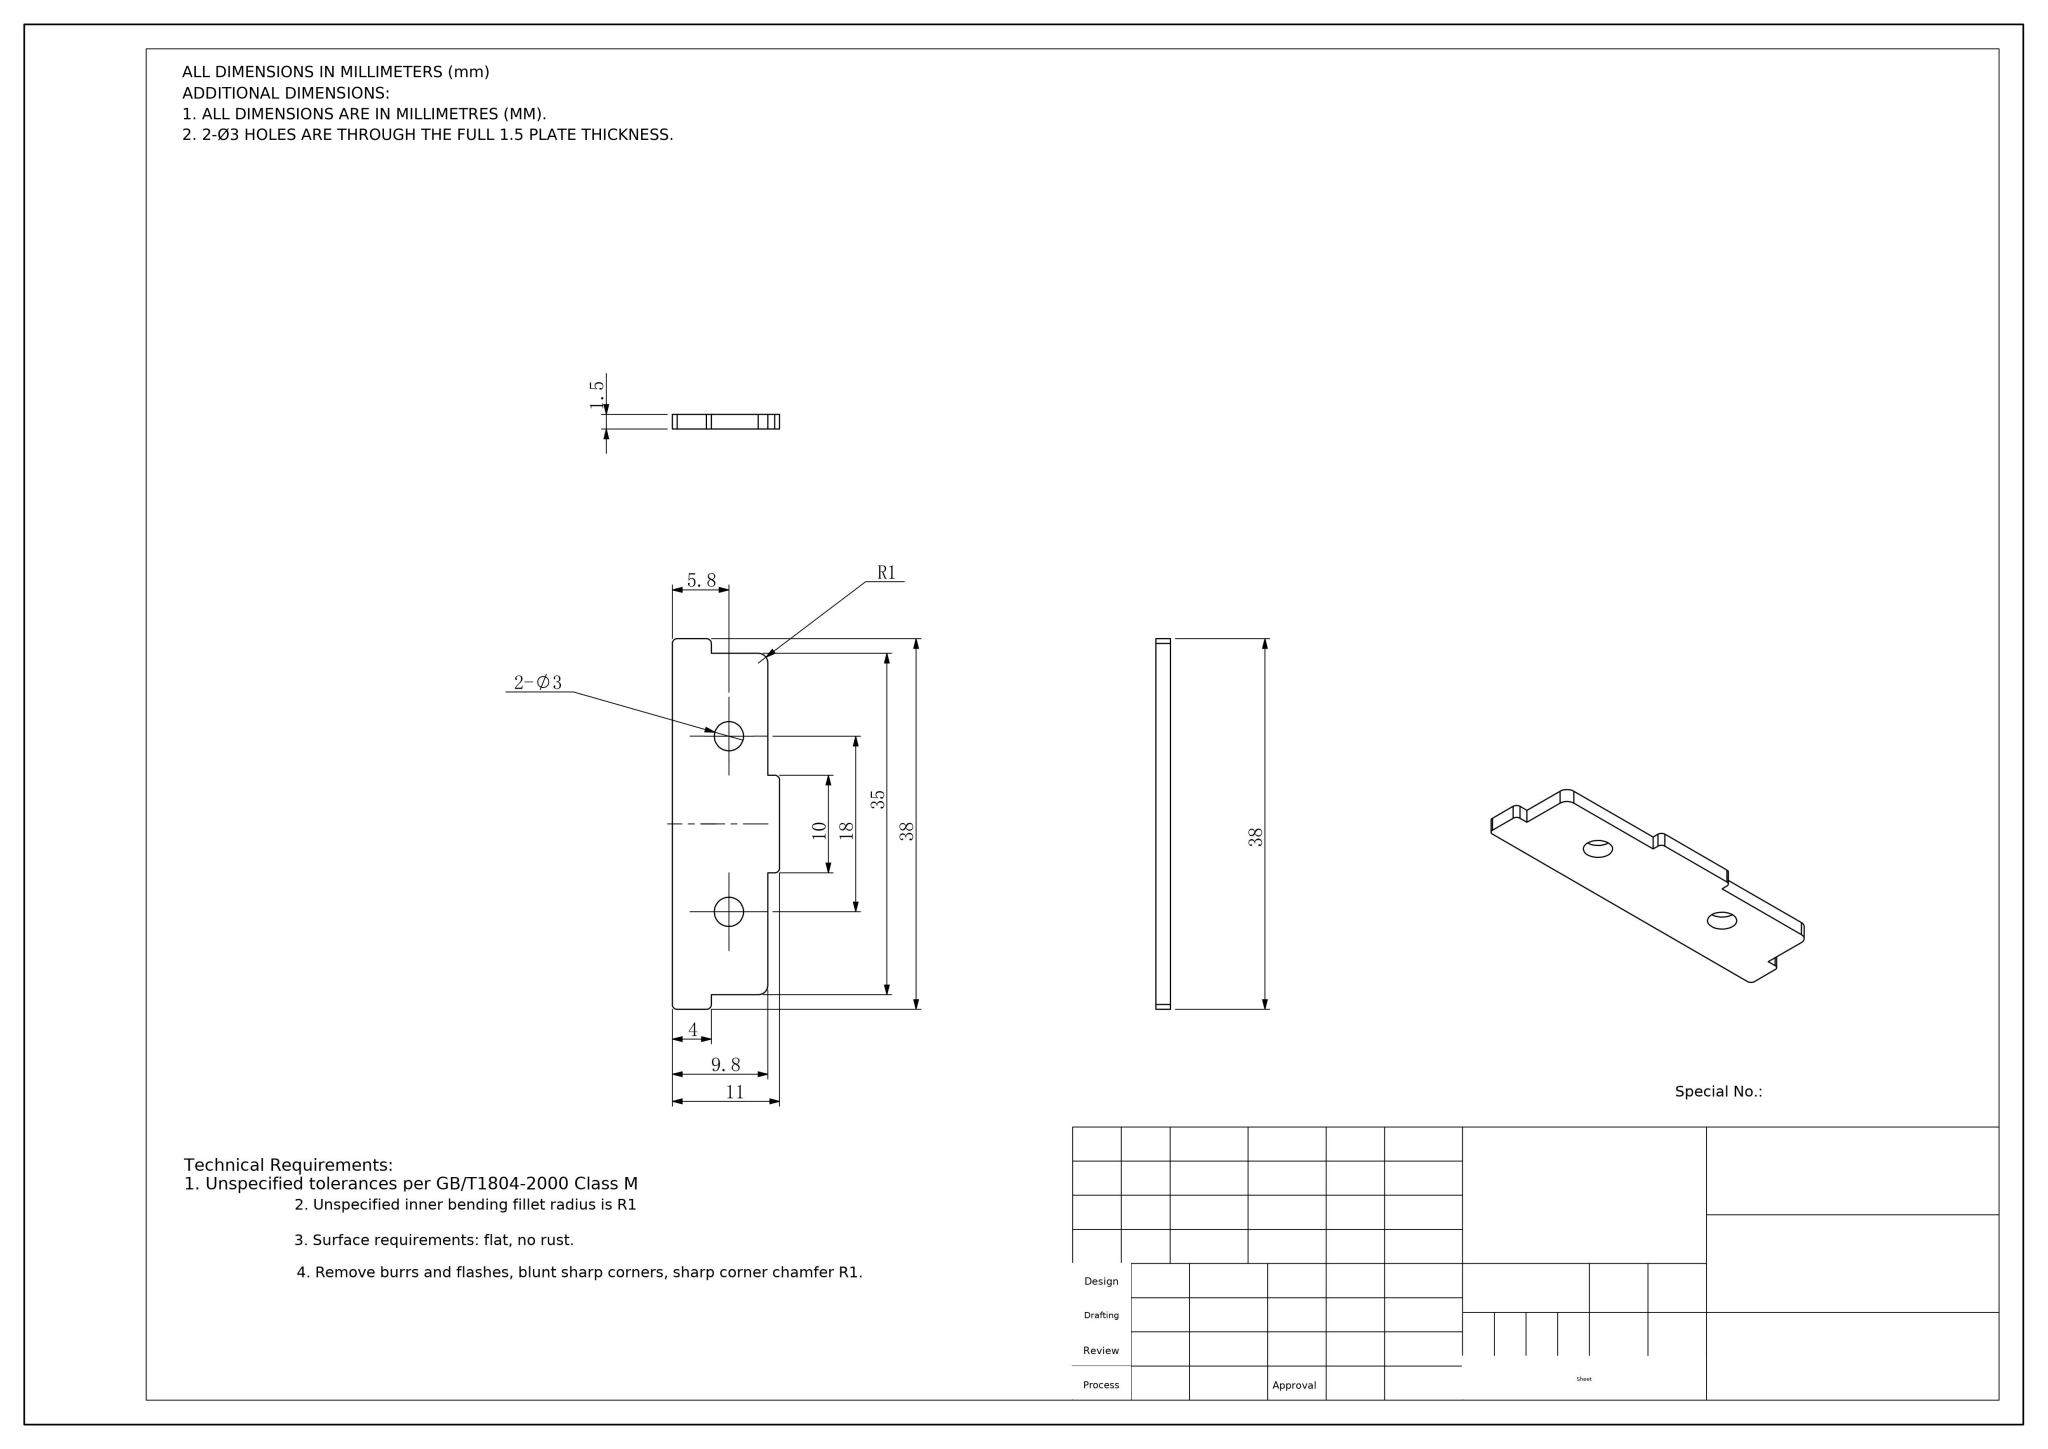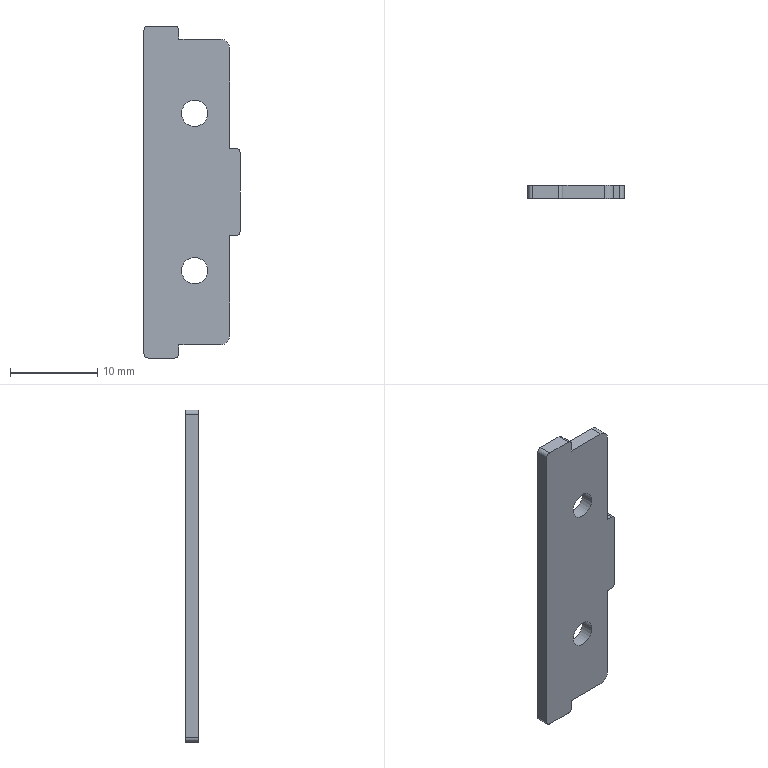Part | NX | mm | Stepped Dual-Bore Mounting Bracket | 1 solid | 26 faces | box 11 x 1.5 x 38 mm | volume 528 mm3 | plane 14 | cylinder 12 | commonest cylinder face diameters 1 x6 3 x4 2 x2
STEP:
#1=COLOUR_RGB('',0.7529,0.7529,0.7529);
#2=FILL_AREA_STYLE_COLOUR('',#1);
#3=FILL_AREA_STYLE('',(#2));
#4=SURFACE_STYLE_FILL_AREA(#3);
#5=SURFACE_SIDE_STYLE('',(#4));
#6=SURFACE_STYLE_USAGE(.BOTH.,#5);
#7=PRESENTATION_STYLE_ASSIGNMENT((#6));
#8=CARTESIAN_POINT('',(-0.2,-1.5,-28.));
#9=VERTEX_POINT('',#8);
#10=CARTESIAN_POINT('',(2.8,-1.5,-28.));
#11=VERTEX_POINT('',#10);
#12=CARTESIAN_POINT('',(1.3,-1.5,-28.));
#13=DIRECTION('',(0.,-1.,0.));
#14=DIRECTION('',(-1.,-0.,0.));
#15=AXIS2_PLACEMENT_3D('',#12,#13,#14);
#16=CIRCLE('',#15,1.5);
#17=EDGE_CURVE('',#9,#11,#16,.T.);
#18=ORIENTED_EDGE('',*,*,#17,.T.);
#19=CARTESIAN_POINT('',(2.8,-0.,-28.));
#20=VERTEX_POINT('',#19);
#21=CARTESIAN_POINT('',(2.8,-0.,-28.));
#22=DIRECTION('',(-0.,1.,0.));
#23=VECTOR('',#22,1000.);
#24=LINE('',#21,#23);
#25=EDGE_CURVE('',#11,#20,#24,.T.);
#26=ORIENTED_EDGE('',*,*,#25,.T.);
#27=CARTESIAN_POINT('',(-0.2,-0.,-28.));
#28=VERTEX_POINT('',#27);
#29=CARTESIAN_POINT('',(1.3,-0.,-28.));
#30=DIRECTION('',(0.,-1.,0.));
#31=DIRECTION('',(-1.,-0.,0.));
#32=AXIS2_PLACEMENT_3D('',#29,#30,#31);
#33=CIRCLE('',#32,1.5);
#34=EDGE_CURVE('',#28,#20,#33,.T.);
#35=ORIENTED_EDGE('',*,*,#34,.F.);
#36=CARTESIAN_POINT('',(-0.2,-0.,-28.));
#37=DIRECTION('',(-0.,1.,0.));
#38=VECTOR('',#37,1000.);
#39=LINE('',#36,#38);
#40=EDGE_CURVE('',#9,#28,#39,.T.);
#41=ORIENTED_EDGE('',*,*,#40,.F.);
#42=EDGE_LOOP('',(#18,#26,#35,#41));
#43=FACE_OUTER_BOUND('',#42,.T.);
#44=CARTESIAN_POINT('',(1.3,-0.,-28.));
#45=DIRECTION('',(-0.,1.,0.));
#46=DIRECTION('',(-1.,-0.,0.));
#47=AXIS2_PLACEMENT_3D('',#44,#45,#46);
#48=CYLINDRICAL_SURFACE('',#47,1.5);
#49=ADVANCED_FACE('',(#43),#48,.F.);
#50=CARTESIAN_POINT('',(-0.2,-1.5,-10.));
#51=VERTEX_POINT('',#50);
#52=CARTESIAN_POINT('',(2.8,-1.5,-10.));
#53=VERTEX_POINT('',#52);
#54=CARTESIAN_POINT('',(1.3,-1.5,-10.));
#55=DIRECTION('',(0.,-1.,0.));
#56=DIRECTION('',(-1.,-0.,0.));
#57=AXIS2_PLACEMENT_3D('',#54,#55,#56);
#58=CIRCLE('',#57,1.5);
#59=EDGE_CURVE('',#51,#53,#58,.T.);
#60=ORIENTED_EDGE('',*,*,#59,.T.);
#61=CARTESIAN_POINT('',(2.8,-0.,-10.));
#62=VERTEX_POINT('',#61);
#63=CARTESIAN_POINT('',(2.8,-0.,-10.));
#64=DIRECTION('',(-0.,1.,0.));
#65=VECTOR('',#64,1000.);
#66=LINE('',#63,#65);
#67=EDGE_CURVE('',#53,#62,#66,.T.);
#68=ORIENTED_EDGE('',*,*,#67,.T.);
#69=CARTESIAN_POINT('',(-0.2,-0.,-10.));
#70=VERTEX_POINT('',#69);
#71=CARTESIAN_POINT('',(1.3,-0.,-10.));
#72=DIRECTION('',(0.,-1.,0.));
#73=DIRECTION('',(-1.,-0.,0.));
#74=AXIS2_PLACEMENT_3D('',#71,#72,#73);
#75=CIRCLE('',#74,1.5);
#76=EDGE_CURVE('',#70,#62,#75,.T.);
#77=ORIENTED_EDGE('',*,*,#76,.F.);
#78=CARTESIAN_POINT('',(-0.2,-0.,-10.));
#79=DIRECTION('',(-0.,1.,0.));
#80=VECTOR('',#79,1000.);
#81=LINE('',#78,#80);
#82=EDGE_CURVE('',#51,#70,#81,.T.);
#83=ORIENTED_EDGE('',*,*,#82,.F.);
#84=EDGE_LOOP('',(#60,#68,#77,#83));
#85=FACE_OUTER_BOUND('',#84,.T.);
#86=CARTESIAN_POINT('',(1.3,-0.,-10.));
#87=DIRECTION('',(-0.,1.,0.));
#88=DIRECTION('',(-1.,-0.,0.));
#89=AXIS2_PLACEMENT_3D('',#86,#87,#88);
#90=CYLINDRICAL_SURFACE('',#89,1.5);
#91=ADVANCED_FACE('',(#85),#90,.F.);
#92=CARTESIAN_POINT('',(-0.5,-1.5,-1.5));
#93=VERTEX_POINT('',#92);
#94=CARTESIAN_POINT('',(4.3,-1.5,-1.5));
#95=VERTEX_POINT('',#94);
#96=CARTESIAN_POINT('',(-4.5,-1.5,-1.5));
#97=DIRECTION('',(1.,0.,0.));
#98=VECTOR('',#97,1000.);
#99=LINE('',#96,#98);
#100=EDGE_CURVE('',#93,#95,#99,.T.);
#101=ORIENTED_EDGE('',*,*,#100,.T.);
#102=CARTESIAN_POINT('',(4.3,-0.,-1.5));
#103=VERTEX_POINT('',#102);
#104=CARTESIAN_POINT('',(4.3,-0.,-1.5));
#105=DIRECTION('',(-0.,1.,0.));
#106=VECTOR('',#105,1000.);
#107=LINE('',#104,#106);
#108=EDGE_CURVE('',#95,#103,#107,.T.);
#109=ORIENTED_EDGE('',*,*,#108,.T.);
#110=CARTESIAN_POINT('',(-0.5,-0.,-1.5));
#111=VERTEX_POINT('',#110);
#112=CARTESIAN_POINT('',(-4.5,-0.,-1.5));
#113=DIRECTION('',(1.,0.,0.));
#114=VECTOR('',#113,1000.);
#115=LINE('',#112,#114);
#116=EDGE_CURVE('',#111,#103,#115,.T.);
#117=ORIENTED_EDGE('',*,*,#116,.F.);
#118=CARTESIAN_POINT('',(-0.5,-0.,-1.5));
#119=DIRECTION('',(0.,-1.,0.));
#120=VECTOR('',#119,1000.);
#121=LINE('',#118,#120);
#122=EDGE_CURVE('',#111,#93,#121,.T.);
#123=ORIENTED_EDGE('',*,*,#122,.T.);
#124=EDGE_LOOP('',(#101,#109,#117,#123));
#125=FACE_OUTER_BOUND('',#124,.T.);
#126=CARTESIAN_POINT('',(-4.5,-0.,-1.5));
#127=DIRECTION('',(0.,0.,1.));
#128=DIRECTION('',(1.,0.,0.));
#129=AXIS2_PLACEMENT_3D('',#126,#127,#128);
#130=PLANE('',#129);
#131=ADVANCED_FACE('',(#125),#130,.T.);
#132=CARTESIAN_POINT('',(-0.5,-0.,-36.5));
#133=VERTEX_POINT('',#132);
#134=CARTESIAN_POINT('',(4.3,-0.,-36.5));
#135=VERTEX_POINT('',#134);
#136=CARTESIAN_POINT('',(-4.5,-0.,-36.5));
#137=DIRECTION('',(1.,0.,0.));
#138=VECTOR('',#137,1000.);
#139=LINE('',#136,#138);
#140=EDGE_CURVE('',#133,#135,#139,.T.);
#141=ORIENTED_EDGE('',*,*,#140,.T.);
#142=CARTESIAN_POINT('',(4.3,-1.5,-36.5));
#143=VERTEX_POINT('',#142);
#144=CARTESIAN_POINT('',(4.3,-0.,-36.5));
#145=DIRECTION('',(0.,-1.,0.));
#146=VECTOR('',#145,1000.);
#147=LINE('',#144,#146);
#148=EDGE_CURVE('',#135,#143,#147,.T.);
#149=ORIENTED_EDGE('',*,*,#148,.T.);
#150=CARTESIAN_POINT('',(-0.5,-1.5,-36.5));
#151=VERTEX_POINT('',#150);
#152=CARTESIAN_POINT('',(-4.5,-1.5,-36.5));
#153=DIRECTION('',(1.,0.,0.));
#154=VECTOR('',#153,1000.);
#155=LINE('',#152,#154);
#156=EDGE_CURVE('',#151,#143,#155,.T.);
#157=ORIENTED_EDGE('',*,*,#156,.F.);
#158=CARTESIAN_POINT('',(-0.5,-0.,-36.5));
#159=DIRECTION('',(-0.,1.,0.));
#160=VECTOR('',#159,1000.);
#161=LINE('',#158,#160);
#162=EDGE_CURVE('',#151,#133,#161,.T.);
#163=ORIENTED_EDGE('',*,*,#162,.T.);
#164=EDGE_LOOP('',(#141,#149,#157,#163));
#165=FACE_OUTER_BOUND('',#164,.T.);
#166=CARTESIAN_POINT('',(-4.5,-0.,-36.5));
#167=DIRECTION('',(0.,0.,1.));
#168=DIRECTION('',(1.,0.,0.));
#169=AXIS2_PLACEMENT_3D('',#166,#167,#168);
#170=PLANE('',#169);
#171=ADVANCED_FACE('',(#165),#170,.F.);
#172=CARTESIAN_POINT('',(5.3,-1.5,-24.));
#173=VERTEX_POINT('',#172);
#174=CARTESIAN_POINT('',(5.3,-1.5,-35.5));
#175=VERTEX_POINT('',#174);
#176=CARTESIAN_POINT('',(5.3,-1.5,-1.3));
#177=DIRECTION('',(0.,0.,-1.));
#178=VECTOR('',#177,1000.);
#179=LINE('',#176,#178);
#180=EDGE_CURVE('',#173,#175,#179,.T.);
#181=ORIENTED_EDGE('',*,*,#180,.T.);
#182=CARTESIAN_POINT('',(5.3,-0.,-35.5));
#183=VERTEX_POINT('',#182);
#184=CARTESIAN_POINT('',(5.3,-0.,-35.5));
#185=DIRECTION('',(-0.,1.,0.));
#186=VECTOR('',#185,1000.);
#187=LINE('',#184,#186);
#188=EDGE_CURVE('',#175,#183,#187,.T.);
#189=ORIENTED_EDGE('',*,*,#188,.T.);
#190=CARTESIAN_POINT('',(5.3,-0.,-24.));
#191=VERTEX_POINT('',#190);
#192=CARTESIAN_POINT('',(5.3,-0.,-1.3));
#193=DIRECTION('',(0.,0.,-1.));
#194=VECTOR('',#193,1000.);
#195=LINE('',#192,#194);
#196=EDGE_CURVE('',#191,#183,#195,.T.);
#197=ORIENTED_EDGE('',*,*,#196,.F.);
#198=CARTESIAN_POINT('',(5.3,-0.,-24.));
#199=DIRECTION('',(0.,-1.,0.));
#200=VECTOR('',#199,1000.);
#201=LINE('',#198,#200);
#202=EDGE_CURVE('',#191,#173,#201,.T.);
#203=ORIENTED_EDGE('',*,*,#202,.T.);
#204=EDGE_LOOP('',(#181,#189,#197,#203));
#205=FACE_OUTER_BOUND('',#204,.T.);
#206=CARTESIAN_POINT('',(5.3,-0.,-1.3));
#207=DIRECTION('',(1.,0.,0.));
#208=DIRECTION('',(0.,0.,-1.));
#209=AXIS2_PLACEMENT_3D('',#206,#207,#208);
#210=PLANE('',#209);
#211=ADVANCED_FACE('',(#205),#210,.T.);
#212=CARTESIAN_POINT('',(5.3,-0.,-2.5));
#213=VERTEX_POINT('',#212);
#214=CARTESIAN_POINT('',(5.3,-0.,-14.));
#215=VERTEX_POINT('',#214);
#216=CARTESIAN_POINT('',(5.3,-0.,-1.3));
#217=DIRECTION('',(0.,0.,-1.));
#218=VECTOR('',#217,1000.);
#219=LINE('',#216,#218);
#220=EDGE_CURVE('',#213,#215,#219,.T.);
#221=ORIENTED_EDGE('',*,*,#220,.F.);
#222=CARTESIAN_POINT('',(5.3,-1.5,-2.5));
#223=VERTEX_POINT('',#222);
#224=CARTESIAN_POINT('',(5.3,-0.,-2.5));
#225=DIRECTION('',(0.,-1.,0.));
#226=VECTOR('',#225,1000.);
#227=LINE('',#224,#226);
#228=EDGE_CURVE('',#213,#223,#227,.T.);
#229=ORIENTED_EDGE('',*,*,#228,.T.);
#230=CARTESIAN_POINT('',(5.3,-1.5,-14.));
#231=VERTEX_POINT('',#230);
#232=CARTESIAN_POINT('',(5.3,-1.5,-1.3));
#233=DIRECTION('',(0.,0.,-1.));
#234=VECTOR('',#233,1000.);
#235=LINE('',#232,#234);
#236=EDGE_CURVE('',#223,#231,#235,.T.);
#237=ORIENTED_EDGE('',*,*,#236,.T.);
#238=CARTESIAN_POINT('',(5.3,-0.,-14.));
#239=DIRECTION('',(-0.,1.,0.));
#240=VECTOR('',#239,1000.);
#241=LINE('',#238,#240);
#242=EDGE_CURVE('',#231,#215,#241,.T.);
#243=ORIENTED_EDGE('',*,*,#242,.T.);
#244=EDGE_LOOP('',(#221,#229,#237,#243));
#245=FACE_OUTER_BOUND('',#244,.T.);
#246=CARTESIAN_POINT('',(5.3,-0.,-1.3));
#247=DIRECTION('',(1.,0.,0.));
#248=DIRECTION('',(0.,0.,-1.));
#249=AXIS2_PLACEMENT_3D('',#246,#247,#248);
#250=PLANE('',#249);
#251=ADVANCED_FACE('',(#245),#250,.T.);
#252=CARTESIAN_POINT('',(-4.5,-0.,-0.5));
#253=VERTEX_POINT('',#252);
#254=CARTESIAN_POINT('',(-4.5,-0.,-37.5));
#255=VERTEX_POINT('',#254);
#256=CARTESIAN_POINT('',(-4.5,-0.,-1.3));
#257=DIRECTION('',(0.,0.,-1.));
#258=VECTOR('',#257,1000.);
#259=LINE('',#256,#258);
#260=EDGE_CURVE('',#253,#255,#259,.T.);
#261=ORIENTED_EDGE('',*,*,#260,.T.);
#262=CARTESIAN_POINT('',(-4.5,-1.5,-37.5));
#263=VERTEX_POINT('',#262);
#264=CARTESIAN_POINT('',(-4.5,-1.5,-37.5));
#265=DIRECTION('',(0.,-1.,0.));
#266=VECTOR('',#265,1000.);
#267=LINE('',#264,#266);
#268=EDGE_CURVE('',#255,#263,#267,.T.);
#269=ORIENTED_EDGE('',*,*,#268,.T.);
#270=CARTESIAN_POINT('',(-4.5,-1.5,-0.5));
#271=VERTEX_POINT('',#270);
#272=CARTESIAN_POINT('',(-4.5,-1.5,-1.3));
#273=DIRECTION('',(0.,0.,-1.));
#274=VECTOR('',#273,1000.);
#275=LINE('',#272,#274);
#276=EDGE_CURVE('',#271,#263,#275,.T.);
#277=ORIENTED_EDGE('',*,*,#276,.F.);
#278=CARTESIAN_POINT('',(-4.5,-0.,-0.5));
#279=DIRECTION('',(-0.,1.,0.));
#280=VECTOR('',#279,1000.);
#281=LINE('',#278,#280);
#282=EDGE_CURVE('',#271,#253,#281,.T.);
#283=ORIENTED_EDGE('',*,*,#282,.T.);
#284=EDGE_LOOP('',(#261,#269,#277,#283));
#285=FACE_OUTER_BOUND('',#284,.T.);
#286=CARTESIAN_POINT('',(-4.5,-0.,-1.3));
#287=DIRECTION('',(1.,0.,0.));
#288=DIRECTION('',(0.,0.,-1.));
#289=AXIS2_PLACEMENT_3D('',#286,#287,#288);
#290=PLANE('',#289);
#291=ADVANCED_FACE('',(#285),#290,.F.);
#292=ORIENTED_EDGE('',*,*,#17,.F.);
#293=CARTESIAN_POINT('',(1.3,-1.5,-28.));
#294=DIRECTION('',(0.,-1.,0.));
#295=DIRECTION('',(-1.,-0.,0.));
#296=AXIS2_PLACEMENT_3D('',#293,#294,#295);
#297=CIRCLE('',#296,1.5);
#298=EDGE_CURVE('',#11,#9,#297,.T.);
#299=ORIENTED_EDGE('',*,*,#298,.F.);
#300=EDGE_LOOP('',(#292,#299));
#301=FACE_BOUND('',#300,.T.);
#302=ORIENTED_EDGE('',*,*,#59,.F.);
#303=CARTESIAN_POINT('',(1.3,-1.5,-10.));
#304=DIRECTION('',(0.,-1.,0.));
#305=DIRECTION('',(-1.,-0.,0.));
#306=AXIS2_PLACEMENT_3D('',#303,#304,#305);
#307=CIRCLE('',#306,1.5);
#308=EDGE_CURVE('',#53,#51,#307,.T.);
#309=ORIENTED_EDGE('',*,*,#308,.F.);
#310=EDGE_LOOP('',(#302,#309));
#311=FACE_BOUND('',#310,.T.);
#312=ORIENTED_EDGE('',*,*,#156,.T.);
#313=CARTESIAN_POINT('',(4.3,-1.5,-35.5));
#314=DIRECTION('',(0.,-1.,0.));
#315=DIRECTION('',(-1.,-0.,0.));
#316=AXIS2_PLACEMENT_3D('',#313,#314,#315);
#317=CIRCLE('',#316,1.);
#318=EDGE_CURVE('',#143,#175,#317,.T.);
#319=ORIENTED_EDGE('',*,*,#318,.T.);
#320=ORIENTED_EDGE('',*,*,#180,.F.);
#321=CARTESIAN_POINT('',(6.,-1.5,-24.));
#322=VERTEX_POINT('',#321);
#323=CARTESIAN_POINT('',(-0.5,-1.5,-24.));
#324=DIRECTION('',(1.,0.,0.));
#325=VECTOR('',#324,1000.);
#326=LINE('',#323,#325);
#327=EDGE_CURVE('',#173,#322,#326,.T.);
#328=ORIENTED_EDGE('',*,*,#327,.T.);
#329=CARTESIAN_POINT('',(6.5,-1.5,-23.5));
#330=VERTEX_POINT('',#329);
#331=CARTESIAN_POINT('',(6.,-1.5,-23.5));
#332=DIRECTION('',(0.,-1.,0.));
#333=DIRECTION('',(-1.,-0.,0.));
#334=AXIS2_PLACEMENT_3D('',#331,#332,#333);
#335=CIRCLE('',#334,0.5);
#336=EDGE_CURVE('',#322,#330,#335,.T.);
#337=ORIENTED_EDGE('',*,*,#336,.T.);
#338=CARTESIAN_POINT('',(6.5,-1.5,-14.5));
#339=VERTEX_POINT('',#338);
#340=CARTESIAN_POINT('',(6.5,-1.5,-14.));
#341=DIRECTION('',(0.,0.,1.));
#342=VECTOR('',#341,1000.);
#343=LINE('',#340,#342);
#344=EDGE_CURVE('',#330,#339,#343,.T.);
#345=ORIENTED_EDGE('',*,*,#344,.T.);
#346=CARTESIAN_POINT('',(6.,-1.5,-14.));
#347=VERTEX_POINT('',#346);
#348=CARTESIAN_POINT('',(6.,-1.5,-14.5));
#349=DIRECTION('',(0.,-1.,0.));
#350=DIRECTION('',(-1.,-0.,0.));
#351=AXIS2_PLACEMENT_3D('',#348,#349,#350);
#352=CIRCLE('',#351,0.5);
#353=EDGE_CURVE('',#339,#347,#352,.T.);
#354=ORIENTED_EDGE('',*,*,#353,.T.);
#355=CARTESIAN_POINT('',(-0.5,-1.5,-14.));
#356=DIRECTION('',(-1.,-0.,0.));
#357=VECTOR('',#356,1000.);
#358=LINE('',#355,#357);
#359=EDGE_CURVE('',#347,#231,#358,.T.);
#360=ORIENTED_EDGE('',*,*,#359,.T.);
#361=ORIENTED_EDGE('',*,*,#236,.F.);
#362=CARTESIAN_POINT('',(4.3,-1.5,-2.5));
#363=DIRECTION('',(0.,-1.,0.));
#364=DIRECTION('',(-1.,-0.,0.));
#365=AXIS2_PLACEMENT_3D('',#362,#363,#364);
#366=CIRCLE('',#365,1.);
#367=EDGE_CURVE('',#223,#95,#366,.T.);
#368=ORIENTED_EDGE('',*,*,#367,.T.);
#369=ORIENTED_EDGE('',*,*,#100,.F.);
#370=CARTESIAN_POINT('',(-0.5,-1.5,-0.5));
#371=VERTEX_POINT('',#370);
#372=CARTESIAN_POINT('',(-0.5,-1.5,0.));
#373=DIRECTION('',(0.,0.,1.));
#374=VECTOR('',#373,1000.);
#375=LINE('',#372,#374);
#376=EDGE_CURVE('',#93,#371,#375,.T.);
#377=ORIENTED_EDGE('',*,*,#376,.T.);
#378=CARTESIAN_POINT('',(-1.,-1.5,0.));
#379=VERTEX_POINT('',#378);
#380=CARTESIAN_POINT('',(-1.,-1.5,-0.5));
#381=DIRECTION('',(0.,-1.,0.));
#382=DIRECTION('',(-1.,-0.,-0.));
#383=AXIS2_PLACEMENT_3D('',#380,#381,#382);
#384=CIRCLE('',#383,0.5);
#385=EDGE_CURVE('',#371,#379,#384,.T.);
#386=ORIENTED_EDGE('',*,*,#385,.T.);
#387=CARTESIAN_POINT('',(-4.,-1.5,0.));
#388=VERTEX_POINT('',#387);
#389=CARTESIAN_POINT('',(-4.5,-1.5,0.));
#390=DIRECTION('',(-1.,-0.,0.));
#391=VECTOR('',#390,1000.);
#392=LINE('',#389,#391);
#393=EDGE_CURVE('',#379,#388,#392,.T.);
#394=ORIENTED_EDGE('',*,*,#393,.T.);
#395=CARTESIAN_POINT('',(-4.,-1.5,-0.5));
#396=DIRECTION('',(0.,-1.,0.));
#397=DIRECTION('',(-1.,-0.,0.));
#398=AXIS2_PLACEMENT_3D('',#395,#396,#397);
#399=CIRCLE('',#398,0.5);
#400=EDGE_CURVE('',#388,#271,#399,.T.);
#401=ORIENTED_EDGE('',*,*,#400,.T.);
#402=ORIENTED_EDGE('',*,*,#276,.T.);
#403=CARTESIAN_POINT('',(-4.,-1.5,-38.));
#404=VERTEX_POINT('',#403);
#405=CARTESIAN_POINT('',(-4.,-1.5,-37.5));
#406=DIRECTION('',(0.,-1.,0.));
#407=DIRECTION('',(-1.,-0.,0.));
#408=AXIS2_PLACEMENT_3D('',#405,#406,#407);
#409=CIRCLE('',#408,0.5);
#410=EDGE_CURVE('',#263,#404,#409,.T.);
#411=ORIENTED_EDGE('',*,*,#410,.T.);
#412=CARTESIAN_POINT('',(-1.,-1.5,-38.));
#413=VERTEX_POINT('',#412);
#414=CARTESIAN_POINT('',(-0.5,-1.5,-38.));
#415=DIRECTION('',(1.,0.,-0.));
#416=VECTOR('',#415,1000.);
#417=LINE('',#414,#416);
#418=EDGE_CURVE('',#404,#413,#417,.T.);
#419=ORIENTED_EDGE('',*,*,#418,.T.);
#420=CARTESIAN_POINT('',(-0.5,-1.5,-37.5));
#421=VERTEX_POINT('',#420);
#422=CARTESIAN_POINT('',(-1.,-1.5,-37.5));
#423=DIRECTION('',(0.,-1.,0.));
#424=DIRECTION('',(-1.,-0.,0.));
#425=AXIS2_PLACEMENT_3D('',#422,#423,#424);
#426=CIRCLE('',#425,0.5);
#427=EDGE_CURVE('',#413,#421,#426,.T.);
#428=ORIENTED_EDGE('',*,*,#427,.T.);
#429=CARTESIAN_POINT('',(-0.5,-1.5,-24.));
#430=DIRECTION('',(0.,0.,1.));
#431=VECTOR('',#430,1000.);
#432=LINE('',#429,#431);
#433=EDGE_CURVE('',#421,#151,#432,.T.);
#434=ORIENTED_EDGE('',*,*,#433,.T.);
#435=EDGE_LOOP('',(#312,#319,#320,#328,#337,#345,#354,#360,#361,#368,#369,#377,#386,#394,#401,#402,#411,#419,#428,#434));
#436=FACE_OUTER_BOUND('',#435,.T.);
#437=CARTESIAN_POINT('',(-4.5,-1.5,-1.3));
#438=DIRECTION('',(-0.,1.,0.));
#439=DIRECTION('',(-1.,-0.,0.));
#440=AXIS2_PLACEMENT_3D('',#437,#438,#439);
#441=PLANE('',#440);
#442=ADVANCED_FACE('',(#301,#311,#436),#441,.F.);
#443=ORIENTED_EDGE('',*,*,#34,.T.);
#444=CARTESIAN_POINT('',(1.3,-0.,-28.));
#445=DIRECTION('',(0.,-1.,0.));
#446=DIRECTION('',(-1.,-0.,0.));
#447=AXIS2_PLACEMENT_3D('',#444,#445,#446);
#448=CIRCLE('',#447,1.5);
#449=EDGE_CURVE('',#20,#28,#448,.T.);
#450=ORIENTED_EDGE('',*,*,#449,.T.);
#451=EDGE_LOOP('',(#443,#450));
#452=FACE_BOUND('',#451,.T.);
#453=ORIENTED_EDGE('',*,*,#76,.T.);
#454=CARTESIAN_POINT('',(1.3,-0.,-10.));
#455=DIRECTION('',(0.,-1.,0.));
#456=DIRECTION('',(-1.,-0.,0.));
#457=AXIS2_PLACEMENT_3D('',#454,#455,#456);
#458=CIRCLE('',#457,1.5);
#459=EDGE_CURVE('',#62,#70,#458,.T.);
#460=ORIENTED_EDGE('',*,*,#459,.T.);
#461=EDGE_LOOP('',(#453,#460));
#462=FACE_BOUND('',#461,.T.);
#463=ORIENTED_EDGE('',*,*,#196,.T.);
#464=CARTESIAN_POINT('',(4.3,-0.,-35.5));
#465=DIRECTION('',(-0.,1.,0.));
#466=DIRECTION('',(-1.,-0.,0.));
#467=AXIS2_PLACEMENT_3D('',#464,#465,#466);
#468=CIRCLE('',#467,1.);
#469=EDGE_CURVE('',#183,#135,#468,.T.);
#470=ORIENTED_EDGE('',*,*,#469,.T.);
#471=ORIENTED_EDGE('',*,*,#140,.F.);
#472=CARTESIAN_POINT('',(-0.5,-0.,-37.5));
#473=VERTEX_POINT('',#472);
#474=CARTESIAN_POINT('',(-0.5,-0.,-24.));
#475=DIRECTION('',(0.,0.,1.));
#476=VECTOR('',#475,1000.);
#477=LINE('',#474,#476);
#478=EDGE_CURVE('',#473,#133,#477,.T.);
#479=ORIENTED_EDGE('',*,*,#478,.F.);
#480=CARTESIAN_POINT('',(-1.,-0.,-38.));
#481=VERTEX_POINT('',#480);
#482=CARTESIAN_POINT('',(-1.,-0.,-37.5));
#483=DIRECTION('',(-0.,1.,0.));
#484=DIRECTION('',(-1.,-0.,0.));
#485=AXIS2_PLACEMENT_3D('',#482,#483,#484);
#486=CIRCLE('',#485,0.5);
#487=EDGE_CURVE('',#473,#481,#486,.T.);
#488=ORIENTED_EDGE('',*,*,#487,.T.);
#489=CARTESIAN_POINT('',(-4.,-0.,-38.));
#490=VERTEX_POINT('',#489);
#491=CARTESIAN_POINT('',(-0.5,-0.,-38.));
#492=DIRECTION('',(1.,0.,-0.));
#493=VECTOR('',#492,1000.);
#494=LINE('',#491,#493);
#495=EDGE_CURVE('',#490,#481,#494,.T.);
#496=ORIENTED_EDGE('',*,*,#495,.F.);
#497=CARTESIAN_POINT('',(-4.,-0.,-37.5));
#498=DIRECTION('',(-0.,1.,0.));
#499=DIRECTION('',(-1.,-0.,0.));
#500=AXIS2_PLACEMENT_3D('',#497,#498,#499);
#501=CIRCLE('',#500,0.5);
#502=EDGE_CURVE('',#490,#255,#501,.T.);
#503=ORIENTED_EDGE('',*,*,#502,.T.);
#504=ORIENTED_EDGE('',*,*,#260,.F.);
#505=CARTESIAN_POINT('',(-4.,-0.,0.));
#506=VERTEX_POINT('',#505);
#507=CARTESIAN_POINT('',(-4.,-0.,-0.5));
#508=DIRECTION('',(-0.,1.,0.));
#509=DIRECTION('',(-1.,-0.,0.));
#510=AXIS2_PLACEMENT_3D('',#507,#508,#509);
#511=CIRCLE('',#510,0.5);
#512=EDGE_CURVE('',#253,#506,#511,.T.);
#513=ORIENTED_EDGE('',*,*,#512,.T.);
#514=CARTESIAN_POINT('',(-1.,-0.,0.));
#515=VERTEX_POINT('',#514);
#516=CARTESIAN_POINT('',(-4.5,-0.,0.));
#517=DIRECTION('',(-1.,-0.,0.));
#518=VECTOR('',#517,1000.);
#519=LINE('',#516,#518);
#520=EDGE_CURVE('',#515,#506,#519,.T.);
#521=ORIENTED_EDGE('',*,*,#520,.F.);
#522=CARTESIAN_POINT('',(-0.5,-0.,-0.5));
#523=VERTEX_POINT('',#522);
#524=CARTESIAN_POINT('',(-1.,-0.,-0.5));
#525=DIRECTION('',(-0.,1.,0.));
#526=DIRECTION('',(-1.,-0.,0.));
#527=AXIS2_PLACEMENT_3D('',#524,#525,#526);
#528=CIRCLE('',#527,0.5);
#529=EDGE_CURVE('',#515,#523,#528,.T.);
#530=ORIENTED_EDGE('',*,*,#529,.T.);
#531=CARTESIAN_POINT('',(-0.5,-0.,0.));
#532=DIRECTION('',(0.,0.,1.));
#533=VECTOR('',#532,1000.);
#534=LINE('',#531,#533);
#535=EDGE_CURVE('',#111,#523,#534,.T.);
#536=ORIENTED_EDGE('',*,*,#535,.F.);
#537=ORIENTED_EDGE('',*,*,#116,.T.);
#538=CARTESIAN_POINT('',(4.3,-0.,-2.5));
#539=DIRECTION('',(-0.,1.,0.));
#540=DIRECTION('',(-1.,-0.,0.));
#541=AXIS2_PLACEMENT_3D('',#538,#539,#540);
#542=CIRCLE('',#541,1.);
#543=EDGE_CURVE('',#103,#213,#542,.T.);
#544=ORIENTED_EDGE('',*,*,#543,.T.);
#545=ORIENTED_EDGE('',*,*,#220,.T.);
#546=CARTESIAN_POINT('',(6.,-0.,-14.));
#547=VERTEX_POINT('',#546);
#548=CARTESIAN_POINT('',(-0.5,-0.,-14.));
#549=DIRECTION('',(-1.,-0.,0.));
#550=VECTOR('',#549,1000.);
#551=LINE('',#548,#550);
#552=EDGE_CURVE('',#547,#215,#551,.T.);
#553=ORIENTED_EDGE('',*,*,#552,.F.);
#554=CARTESIAN_POINT('',(6.5,-0.,-14.5));
#555=VERTEX_POINT('',#554);
#556=CARTESIAN_POINT('',(6.,-0.,-14.5));
#557=DIRECTION('',(-0.,1.,0.));
#558=DIRECTION('',(-1.,-0.,0.));
#559=AXIS2_PLACEMENT_3D('',#556,#557,#558);
#560=CIRCLE('',#559,0.5);
#561=EDGE_CURVE('',#547,#555,#560,.T.);
#562=ORIENTED_EDGE('',*,*,#561,.T.);
#563=CARTESIAN_POINT('',(6.5,-0.,-23.5));
#564=VERTEX_POINT('',#563);
#565=CARTESIAN_POINT('',(6.5,-0.,-14.));
#566=DIRECTION('',(0.,0.,1.));
#567=VECTOR('',#566,1000.);
#568=LINE('',#565,#567);
#569=EDGE_CURVE('',#564,#555,#568,.T.);
#570=ORIENTED_EDGE('',*,*,#569,.F.);
#571=CARTESIAN_POINT('',(6.,-0.,-24.));
#572=VERTEX_POINT('',#571);
#573=CARTESIAN_POINT('',(6.,-0.,-23.5));
#574=DIRECTION('',(-0.,1.,0.));
#575=DIRECTION('',(-1.,-0.,0.));
#576=AXIS2_PLACEMENT_3D('',#573,#574,#575);
#577=CIRCLE('',#576,0.5);
#578=EDGE_CURVE('',#564,#572,#577,.T.);
#579=ORIENTED_EDGE('',*,*,#578,.T.);
#580=CARTESIAN_POINT('',(-0.5,-0.,-24.));
#581=DIRECTION('',(1.,0.,0.));
#582=VECTOR('',#581,1000.);
#583=LINE('',#580,#582);
#584=EDGE_CURVE('',#191,#572,#583,.T.);
#585=ORIENTED_EDGE('',*,*,#584,.F.);
#586=EDGE_LOOP('',(#463,#470,#471,#479,#488,#496,#503,#504,#513,#521,#530,#536,#537,#544,#545,#553,#562,#570,#579,#585));
#587=FACE_OUTER_BOUND('',#586,.T.);
#588=CARTESIAN_POINT('',(-4.5,-0.,-1.3));
#589=DIRECTION('',(-0.,1.,0.));
#590=DIRECTION('',(-1.,-0.,0.));
#591=AXIS2_PLACEMENT_3D('',#588,#589,#590);
#592=PLANE('',#591);
#593=ADVANCED_FACE('',(#452,#462,#587),#592,.T.);
#594=ORIENTED_EDGE('',*,*,#344,.F.);
#595=CARTESIAN_POINT('',(6.5,-1.5,-23.5));
#596=DIRECTION('',(-0.,1.,0.));
#597=VECTOR('',#596,1000.);
#598=LINE('',#595,#597);
#599=EDGE_CURVE('',#330,#564,#598,.T.);
#600=ORIENTED_EDGE('',*,*,#599,.T.);
#601=ORIENTED_EDGE('',*,*,#569,.T.);
#602=CARTESIAN_POINT('',(6.5,-1.5,-14.5));
#603=DIRECTION('',(0.,-1.,0.));
#604=VECTOR('',#603,1000.);
#605=LINE('',#602,#604);
#606=EDGE_CURVE('',#555,#339,#605,.T.);
#607=ORIENTED_EDGE('',*,*,#606,.T.);
#608=EDGE_LOOP('',(#594,#600,#601,#607));
#609=FACE_OUTER_BOUND('',#608,.T.);
#610=CARTESIAN_POINT('',(6.5,-1.5,-14.));
#611=DIRECTION('',(-1.,-0.,0.));
#612=DIRECTION('',(0.,0.,1.));
#613=AXIS2_PLACEMENT_3D('',#610,#611,#612);
#614=PLANE('',#613);
#615=ADVANCED_FACE('',(#609),#614,.F.);
#616=ORIENTED_EDGE('',*,*,#359,.F.);
#617=CARTESIAN_POINT('',(6.,-1.5,-14.));
#618=DIRECTION('',(-0.,1.,0.));
#619=VECTOR('',#618,1000.);
#620=LINE('',#617,#619);
#621=EDGE_CURVE('',#347,#547,#620,.T.);
#622=ORIENTED_EDGE('',*,*,#621,.T.);
#623=ORIENTED_EDGE('',*,*,#552,.T.);
#624=ORIENTED_EDGE('',*,*,#242,.F.);
#625=EDGE_LOOP('',(#616,#622,#623,#624));
#626=FACE_OUTER_BOUND('',#625,.T.);
#627=CARTESIAN_POINT('',(-0.5,-1.5,-14.));
#628=DIRECTION('',(0.,0.,-1.));
#629=DIRECTION('',(-1.,0.,0.));
#630=AXIS2_PLACEMENT_3D('',#627,#628,#629);
#631=PLANE('',#630);
#632=ADVANCED_FACE('',(#626),#631,.F.);
#633=ORIENTED_EDGE('',*,*,#584,.T.);
#634=CARTESIAN_POINT('',(6.,-1.5,-24.));
#635=DIRECTION('',(0.,-1.,0.));
#636=VECTOR('',#635,1000.);
#637=LINE('',#634,#636);
#638=EDGE_CURVE('',#572,#322,#637,.T.);
#639=ORIENTED_EDGE('',*,*,#638,.T.);
#640=ORIENTED_EDGE('',*,*,#327,.F.);
#641=ORIENTED_EDGE('',*,*,#202,.F.);
#642=EDGE_LOOP('',(#633,#639,#640,#641));
#643=FACE_OUTER_BOUND('',#642,.T.);
#644=CARTESIAN_POINT('',(-0.5,-1.5,-24.));
#645=DIRECTION('',(0.,0.,1.));
#646=DIRECTION('',(1.,0.,0.));
#647=AXIS2_PLACEMENT_3D('',#644,#645,#646);
#648=PLANE('',#647);
#649=ADVANCED_FACE('',(#643),#648,.F.);
#650=ORIENTED_EDGE('',*,*,#495,.T.);
#651=CARTESIAN_POINT('',(-1.,-1.5,-38.));
#652=DIRECTION('',(0.,-1.,0.));
#653=VECTOR('',#652,1000.);
#654=LINE('',#651,#653);
#655=EDGE_CURVE('',#481,#413,#654,.T.);
#656=ORIENTED_EDGE('',*,*,#655,.T.);
#657=ORIENTED_EDGE('',*,*,#418,.F.);
#658=CARTESIAN_POINT('',(-4.,-0.,-38.));
#659=DIRECTION('',(-0.,1.,0.));
#660=VECTOR('',#659,1000.);
#661=LINE('',#658,#660);
#662=EDGE_CURVE('',#404,#490,#661,.T.);
#663=ORIENTED_EDGE('',*,*,#662,.T.);
#664=EDGE_LOOP('',(#650,#656,#657,#663));
#665=FACE_OUTER_BOUND('',#664,.T.);
#666=CARTESIAN_POINT('',(-0.5,-1.5,-38.));
#667=DIRECTION('',(0.,0.,1.));
#668=DIRECTION('',(1.,0.,-0.));
#669=AXIS2_PLACEMENT_3D('',#666,#667,#668);
#670=PLANE('',#669);
#671=ADVANCED_FACE('',(#665),#670,.F.);
#672=ORIENTED_EDGE('',*,*,#433,.F.);
#673=CARTESIAN_POINT('',(-0.5,-1.5,-37.5));
#674=DIRECTION('',(-0.,1.,0.));
#675=VECTOR('',#674,1000.);
#676=LINE('',#673,#675);
#677=EDGE_CURVE('',#421,#473,#676,.T.);
#678=ORIENTED_EDGE('',*,*,#677,.T.);
#679=ORIENTED_EDGE('',*,*,#478,.T.);
#680=ORIENTED_EDGE('',*,*,#162,.F.);
#681=EDGE_LOOP('',(#672,#678,#679,#680));
#682=FACE_OUTER_BOUND('',#681,.T.);
#683=CARTESIAN_POINT('',(-0.5,-1.5,-24.));
#684=DIRECTION('',(-1.,-0.,0.));
#685=DIRECTION('',(0.,-1.,0.));
#686=AXIS2_PLACEMENT_3D('',#683,#684,#685);
#687=PLANE('',#686);
#688=ADVANCED_FACE('',(#682),#687,.F.);
#689=ORIENTED_EDGE('',*,*,#535,.T.);
#690=CARTESIAN_POINT('',(-0.5,-1.5,-0.5));
#691=DIRECTION('',(0.,-1.,0.));
#692=VECTOR('',#691,1000.);
#693=LINE('',#690,#692);
#694=EDGE_CURVE('',#523,#371,#693,.T.);
#695=ORIENTED_EDGE('',*,*,#694,.T.);
#696=ORIENTED_EDGE('',*,*,#376,.F.);
#697=ORIENTED_EDGE('',*,*,#122,.F.);
#698=EDGE_LOOP('',(#689,#695,#696,#697));
#699=FACE_OUTER_BOUND('',#698,.T.);
#700=CARTESIAN_POINT('',(-0.5,-1.5,0.));
#701=DIRECTION('',(-1.,-0.,0.));
#702=DIRECTION('',(0.,-1.,0.));
#703=AXIS2_PLACEMENT_3D('',#700,#701,#702);
#704=PLANE('',#703);
#705=ADVANCED_FACE('',(#699),#704,.F.);
#706=ORIENTED_EDGE('',*,*,#393,.F.);
#707=CARTESIAN_POINT('',(-1.,-1.5,0.));
#708=DIRECTION('',(-0.,1.,0.));
#709=VECTOR('',#708,1000.);
#710=LINE('',#707,#709);
#711=EDGE_CURVE('',#379,#515,#710,.T.);
#712=ORIENTED_EDGE('',*,*,#711,.T.);
#713=ORIENTED_EDGE('',*,*,#520,.T.);
#714=CARTESIAN_POINT('',(-4.,-1.5,0.));
#715=DIRECTION('',(0.,-1.,0.));
#716=VECTOR('',#715,1000.);
#717=LINE('',#714,#716);
#718=EDGE_CURVE('',#506,#388,#717,.T.);
#719=ORIENTED_EDGE('',*,*,#718,.T.);
#720=EDGE_LOOP('',(#706,#712,#713,#719));
#721=FACE_OUTER_BOUND('',#720,.T.);
#722=CARTESIAN_POINT('',(-4.5,-1.5,0.));
#723=DIRECTION('',(-0.,-0.,-1.));
#724=DIRECTION('',(-1.,0.,0.));
#725=AXIS2_PLACEMENT_3D('',#722,#723,#724);
#726=PLANE('',#725);
#727=ADVANCED_FACE('',(#721),#726,.F.);
#728=ORIENTED_EDGE('',*,*,#336,.F.);
#729=ORIENTED_EDGE('',*,*,#638,.F.);
#730=ORIENTED_EDGE('',*,*,#578,.F.);
#731=ORIENTED_EDGE('',*,*,#599,.F.);
#732=EDGE_LOOP('',(#728,#729,#730,#731));
#733=FACE_OUTER_BOUND('',#732,.T.);
#734=CARTESIAN_POINT('',(6.,-1.5,-23.5));
#735=DIRECTION('',(-0.,1.,0.));
#736=DIRECTION('',(-1.,-0.,0.));
#737=AXIS2_PLACEMENT_3D('',#734,#735,#736);
#738=CYLINDRICAL_SURFACE('',#737,0.5);
#739=ADVANCED_FACE('',(#733),#738,.T.);
#740=ORIENTED_EDGE('',*,*,#353,.F.);
#741=ORIENTED_EDGE('',*,*,#606,.F.);
#742=ORIENTED_EDGE('',*,*,#561,.F.);
#743=ORIENTED_EDGE('',*,*,#621,.F.);
#744=EDGE_LOOP('',(#740,#741,#742,#743));
#745=FACE_OUTER_BOUND('',#744,.T.);
#746=CARTESIAN_POINT('',(6.,-1.5,-14.5));
#747=DIRECTION('',(-0.,1.,0.));
#748=DIRECTION('',(-1.,-0.,0.));
#749=AXIS2_PLACEMENT_3D('',#746,#747,#748);
#750=CYLINDRICAL_SURFACE('',#749,0.5);
#751=ADVANCED_FACE('',(#745),#750,.T.);
#752=ORIENTED_EDGE('',*,*,#427,.F.);
#753=ORIENTED_EDGE('',*,*,#655,.F.);
#754=ORIENTED_EDGE('',*,*,#487,.F.);
#755=ORIENTED_EDGE('',*,*,#677,.F.);
#756=EDGE_LOOP('',(#752,#753,#754,#755));
#757=FACE_OUTER_BOUND('',#756,.T.);
#758=CARTESIAN_POINT('',(-1.,-1.5,-37.5));
#759=DIRECTION('',(-0.,1.,0.));
#760=DIRECTION('',(-1.,-0.,0.));
#761=AXIS2_PLACEMENT_3D('',#758,#759,#760);
#762=CYLINDRICAL_SURFACE('',#761,0.5);
#763=ADVANCED_FACE('',(#757),#762,.T.);
#764=ORIENTED_EDGE('',*,*,#410,.F.);
#765=ORIENTED_EDGE('',*,*,#268,.F.);
#766=ORIENTED_EDGE('',*,*,#502,.F.);
#767=ORIENTED_EDGE('',*,*,#662,.F.);
#768=EDGE_LOOP('',(#764,#765,#766,#767));
#769=FACE_OUTER_BOUND('',#768,.T.);
#770=CARTESIAN_POINT('',(-4.,-1.5,-37.5));
#771=DIRECTION('',(-0.,1.,0.));
#772=DIRECTION('',(-1.,-0.,0.));
#773=AXIS2_PLACEMENT_3D('',#770,#771,#772);
#774=CYLINDRICAL_SURFACE('',#773,0.5);
#775=ADVANCED_FACE('',(#769),#774,.T.);
#776=ORIENTED_EDGE('',*,*,#385,.F.);
#777=ORIENTED_EDGE('',*,*,#694,.F.);
#778=ORIENTED_EDGE('',*,*,#529,.F.);
#779=ORIENTED_EDGE('',*,*,#711,.F.);
#780=EDGE_LOOP('',(#776,#777,#778,#779));
#781=FACE_OUTER_BOUND('',#780,.T.);
#782=CARTESIAN_POINT('',(-1.,-1.5,-0.5));
#783=DIRECTION('',(-0.,1.,0.));
#784=DIRECTION('',(-1.,-0.,0.));
#785=AXIS2_PLACEMENT_3D('',#782,#783,#784);
#786=CYLINDRICAL_SURFACE('',#785,0.5);
#787=ADVANCED_FACE('',(#781),#786,.T.);
#788=ORIENTED_EDGE('',*,*,#400,.F.);
#789=ORIENTED_EDGE('',*,*,#718,.F.);
#790=ORIENTED_EDGE('',*,*,#512,.F.);
#791=ORIENTED_EDGE('',*,*,#282,.F.);
#792=EDGE_LOOP('',(#788,#789,#790,#791));
#793=FACE_OUTER_BOUND('',#792,.T.);
#794=CARTESIAN_POINT('',(-4.,-0.,-0.5));
#795=DIRECTION('',(-0.,1.,0.));
#796=DIRECTION('',(-1.,-0.,0.));
#797=AXIS2_PLACEMENT_3D('',#794,#795,#796);
#798=CYLINDRICAL_SURFACE('',#797,0.5);
#799=ADVANCED_FACE('',(#793),#798,.T.);
#800=ORIENTED_EDGE('',*,*,#469,.F.);
#801=ORIENTED_EDGE('',*,*,#188,.F.);
#802=ORIENTED_EDGE('',*,*,#318,.F.);
#803=ORIENTED_EDGE('',*,*,#148,.F.);
#804=EDGE_LOOP('',(#800,#801,#802,#803));
#805=FACE_OUTER_BOUND('',#804,.T.);
#806=CARTESIAN_POINT('',(4.3,-0.,-35.5));
#807=DIRECTION('',(-0.,1.,0.));
#808=DIRECTION('',(-1.,-0.,0.));
#809=AXIS2_PLACEMENT_3D('',#806,#807,#808);
#810=CYLINDRICAL_SURFACE('',#809,1.);
#811=ADVANCED_FACE('',(#805),#810,.T.);
#812=ORIENTED_EDGE('',*,*,#543,.F.);
#813=ORIENTED_EDGE('',*,*,#108,.F.);
#814=ORIENTED_EDGE('',*,*,#367,.F.);
#815=ORIENTED_EDGE('',*,*,#228,.F.);
#816=EDGE_LOOP('',(#812,#813,#814,#815));
#817=FACE_OUTER_BOUND('',#816,.T.);
#818=CARTESIAN_POINT('',(4.3,-0.,-2.5));
#819=DIRECTION('',(0.,-1.,0.));
#820=DIRECTION('',(1.,0.,0.));
#821=AXIS2_PLACEMENT_3D('',#818,#819,#820);
#822=CYLINDRICAL_SURFACE('',#821,1.);
#823=ADVANCED_FACE('',(#817),#822,.T.);
#824=ORIENTED_EDGE('',*,*,#67,.F.);
#825=ORIENTED_EDGE('',*,*,#308,.T.);
#826=ORIENTED_EDGE('',*,*,#82,.T.);
#827=ORIENTED_EDGE('',*,*,#459,.F.);
#828=EDGE_LOOP('',(#824,#825,#826,#827));
#829=FACE_OUTER_BOUND('',#828,.T.);
#830=CARTESIAN_POINT('',(1.3,-0.,-10.));
#831=DIRECTION('',(-0.,1.,0.));
#832=DIRECTION('',(-1.,-0.,0.));
#833=AXIS2_PLACEMENT_3D('',#830,#831,#832);
#834=CYLINDRICAL_SURFACE('',#833,1.5);
#835=ADVANCED_FACE('',(#829),#834,.F.);
#836=ORIENTED_EDGE('',*,*,#25,.F.);
#837=ORIENTED_EDGE('',*,*,#298,.T.);
#838=ORIENTED_EDGE('',*,*,#40,.T.);
#839=ORIENTED_EDGE('',*,*,#449,.F.);
#840=EDGE_LOOP('',(#836,#837,#838,#839));
#841=FACE_OUTER_BOUND('',#840,.T.);
#842=CARTESIAN_POINT('',(1.3,-0.,-28.));
#843=DIRECTION('',(-0.,1.,0.));
#844=DIRECTION('',(-1.,-0.,0.));
#845=AXIS2_PLACEMENT_3D('',#842,#843,#844);
#846=CYLINDRICAL_SURFACE('',#845,1.5);
#847=ADVANCED_FACE('',(#841),#846,.F.);
#848=CLOSED_SHELL('',(#49,#91,#131,#171,#211,#251,#291,#442,#593,#615,#632,#649,#671,#688,#705,#727,#739,#751,#763,#775,#787,#799,#811,#823,#835,#847));
#849=MANIFOLD_SOLID_BREP('',#848);
#850=CARTESIAN_POINT('',(0.,0.,0.));
#851=DIRECTION('',(0.,0.,1.));
#852=DIRECTION('',(1.,0.,0.));
#853=AXIS2_PLACEMENT_3D('',#850,#851,#852);
#854=(LENGTH_UNIT()NAMED_UNIT(*)SI_UNIT(.MILLI.,.METRE.));
#855=UNCERTAINTY_MEASURE_WITH_UNIT(LENGTH_MEASURE(0.00001),#854,'','');
#856=(NAMED_UNIT(*)PLANE_ANGLE_UNIT()SI_UNIT($,.RADIAN.));
#857=(NAMED_UNIT(*)SI_UNIT($,.STERADIAN.)SOLID_ANGLE_UNIT());
#858=(GEOMETRIC_REPRESENTATION_CONTEXT(3)GLOBAL_UNCERTAINTY_ASSIGNED_CONTEXT((#855))GLOBAL_UNIT_ASSIGNED_CONTEXT((#854,#856,#857))REPRESENTATION_CONTEXT('',''));
#859=ADVANCED_BREP_SHAPE_REPRESENTATION('',(#849,#853),#858);
#860=STYLED_ITEM('',(#7),#859);
#861=(LENGTH_UNIT()NAMED_UNIT(*)SI_UNIT(.MILLI.,.METRE.));
#862=UNCERTAINTY_MEASURE_WITH_UNIT(LENGTH_MEASURE(0.00001),#861,'','');
#863=(NAMED_UNIT(*)PLANE_ANGLE_UNIT()SI_UNIT($,.RADIAN.));
#864=(NAMED_UNIT(*)SI_UNIT($,.STERADIAN.)SOLID_ANGLE_UNIT());
#865=(GEOMETRIC_REPRESENTATION_CONTEXT(3)GLOBAL_UNCERTAINTY_ASSIGNED_CONTEXT((#862))GLOBAL_UNIT_ASSIGNED_CONTEXT((#861,#863,#864))REPRESENTATION_CONTEXT('',''));
#866=MECHANICAL_DESIGN_GEOMETRIC_PRESENTATION_REPRESENTATION('',(#860),#865);
#867=PRESENTATION_LAYER_ASSIGNMENT('','',(#860));
#868=COLOUR_RGB('',0.7529,0.7529,0.7529);
#869=FILL_AREA_STYLE_COLOUR('',#868);
#870=FILL_AREA_STYLE('',(#869));
#871=SURFACE_STYLE_FILL_AREA(#870);
#872=SURFACE_SIDE_STYLE('',(#871));
#873=SURFACE_STYLE_USAGE(.BOTH.,#872);
#874=PRESENTATION_STYLE_ASSIGNMENT((#873));
#875=STYLED_ITEM('',(#874),#849);
#876=(LENGTH_UNIT()NAMED_UNIT(*)SI_UNIT(.MILLI.,.METRE.));
#877=UNCERTAINTY_MEASURE_WITH_UNIT(LENGTH_MEASURE(0.00001),#876,'','');
#878=(NAMED_UNIT(*)PLANE_ANGLE_UNIT()SI_UNIT($,.RADIAN.));
#879=(NAMED_UNIT(*)SI_UNIT($,.STERADIAN.)SOLID_ANGLE_UNIT());
#880=(GEOMETRIC_REPRESENTATION_CONTEXT(3)GLOBAL_UNCERTAINTY_ASSIGNED_CONTEXT((#877))GLOBAL_UNIT_ASSIGNED_CONTEXT((#876,#878,#879))REPRESENTATION_CONTEXT('',''));
#881=MECHANICAL_DESIGN_GEOMETRIC_PRESENTATION_REPRESENTATION('',(#875),#880);
#882=PRESENTATION_LAYER_ASSIGNMENT('','',(#875));